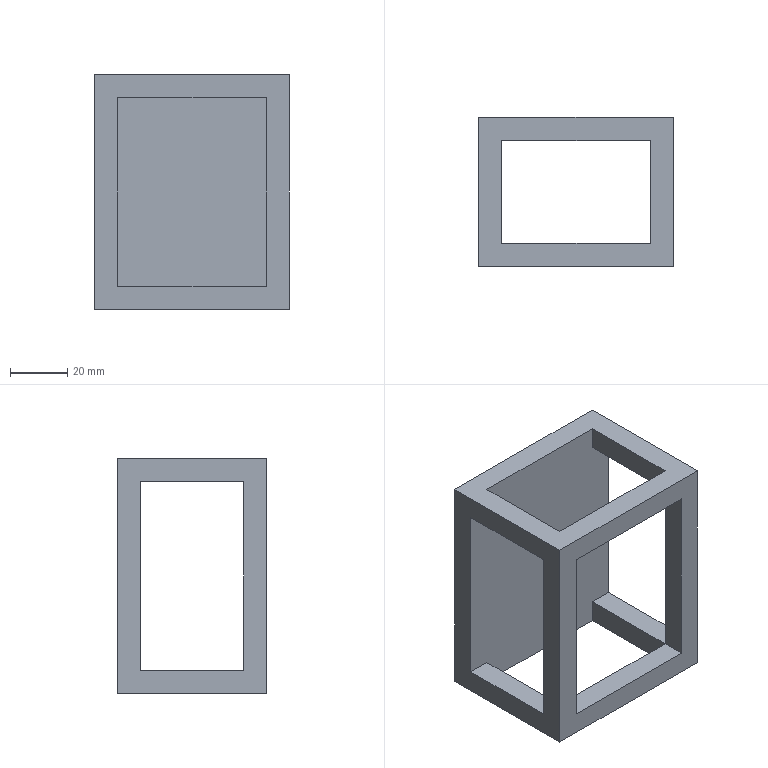Component | SolidWorks | MotorMount-1 | 1 solid | 23 faces | box 68 x 52 x 82 mm | volume 70976 mm3 | plane 23
build123d program:
from build123d import *

# Parameters (mm, degrees)
SKETCH1_W           = 82
SKETCH1_H           = 68
BOSS_EXTRUDE1_DEPTH = 52
SKETCH2_W           = 36
SKETCH2_H           = 52
CUT_EXTRUDE1_DEPTH  = 82
CUT_EXTRUDE2_REACH  = 96.916
SKETCH3_W           = 66
SKETCH3_H           = 36
SKETCH4_W           = 66
SKETCH4_H           = 52
CUT_EXTRUDE3_DEPTH  = 44


with BuildPart() as part:
    # Sketch1 → Boss-Extrude1 (new body)
    with BuildSketch(Plane.XY):
        Rectangle(SKETCH1_W, SKETCH1_H)
    extrude(amount=BOSS_EXTRUDE1_DEPTH)

    # Sketch2 → Cut-Extrude1 (cut)
    with BuildSketch(Plane(origin=(41, 0, 0), x_dir=(0, 0, -1), z_dir=(1, 0, 0))):
        with Locations((-26, 0)):
            Rectangle(SKETCH2_W, SKETCH2_H)
    extrude(amount=-CUT_EXTRUDE1_DEPTH, mode=Mode.SUBTRACT)

    # Cut-Extrude2: up to this face of the body (flat: up to its plane)
    cut_extrude2_end = Plane(part.part.faces().sort_by_distance((0, -34, 26))[0])
    # Sketch3 → Cut-Extrude2 (cut, up to the picked face)
    with BuildSketch(Plane(origin=(0, 34, 0), x_dir=(1, 0, 0), z_dir=(0, 1, 0)), mode=Mode.PRIVATE) as cut_extrude2_sk1:
        with Locations((0, -26)):
            Rectangle(SKETCH3_W, SKETCH3_H)
    cut_extrude2_tool1 = split(extrude(cut_extrude2_sk1.sketch, amount=-CUT_EXTRUDE2_REACH, mode=Mode.PRIVATE), bisect_by=cut_extrude2_end, keep=Keep.BOTH, mode=Mode.PRIVATE)
    add(cut_extrude2_tool1.solids().sort_by(Axis((0, 34, 26), (0, -1, 0)))[0], mode=Mode.SUBTRACT)

    # Sketch4 → Cut-Extrude3 (cut)
    with BuildSketch(Plane.XY.offset(52)):
        Rectangle(SKETCH4_W, SKETCH4_H)
    extrude(amount=-CUT_EXTRUDE3_DEPTH, mode=Mode.SUBTRACT)


solid = part.part

# Placed as in the assembly
solid = solid.moved(Location((-613.2, 52, 0), (90, 0, 90)))
STEP:
#1=CARTESIAN_POINT('',(-25.165,0.315,1.299));
#2=VERTEX_POINT('',#1);
#3=CARTESIAN_POINT('',(-25.48,0.315,1.299));
#4=VERTEX_POINT('',#3);
#5=CARTESIAN_POINT('',(-19.843,0.315,1.299));
#6=DIRECTION('',(-1.,0.,0.));
#7=VECTOR('',#6,39.37);
#8=LINE('',#5,#7);
#9=EDGE_CURVE('',#2,#4,#8,.T.);
#10=ORIENTED_EDGE('',*,*,#9,.F.);
#11=CARTESIAN_POINT('',(-25.165,0.315,-1.299));
#12=VERTEX_POINT('',#11);
#13=CARTESIAN_POINT('',(-25.165,0.315,-4.104));
#14=DIRECTION('',(-0.,0.,-1.));
#15=VECTOR('',#14,39.37);
#16=LINE('',#13,#15);
#17=EDGE_CURVE('',#2,#12,#16,.T.);
#18=ORIENTED_EDGE('',*,*,#17,.T.);
#19=CARTESIAN_POINT('',(-25.48,0.315,-1.299));
#20=VERTEX_POINT('',#19);
#21=CARTESIAN_POINT('',(-19.843,0.315,-1.299));
#22=DIRECTION('',(-1.,0.,0.));
#23=VECTOR('',#22,39.37);
#24=LINE('',#21,#23);
#25=EDGE_CURVE('',#12,#20,#24,.T.);
#26=ORIENTED_EDGE('',*,*,#25,.T.);
#27=CARTESIAN_POINT('',(-25.48,0.315,-1.299));
#28=DIRECTION('',(0.,-0.,1.));
#29=VECTOR('',#28,39.37);
#30=LINE('',#27,#29);
#31=EDGE_CURVE('',#20,#4,#30,.T.);
#32=ORIENTED_EDGE('',*,*,#31,.T.);
#33=EDGE_LOOP('',(#10,#18,#26,#32));
#34=FACE_OUTER_BOUND('',#33,.T.);
#35=CARTESIAN_POINT('',(-25.165,0.315,-4.104));
#36=DIRECTION('',(-0.,-1.,-0.));
#37=DIRECTION('',(0.,-0.,1.));
#38=AXIS2_PLACEMENT_3D('',#35,#36,#37);
#39=PLANE('',#38);
#40=ADVANCED_FACE('',(#34),#39,.F.);
#41=CARTESIAN_POINT('',(-25.165,0.315,-1.614));
#42=VERTEX_POINT('',#41);
#43=CARTESIAN_POINT('',(-25.165,0.315,-4.104));
#44=DIRECTION('',(0.,-0.,1.));
#45=VECTOR('',#44,39.37);
#46=LINE('',#43,#45);
#47=EDGE_CURVE('',#42,#12,#46,.T.);
#48=ORIENTED_EDGE('',*,*,#47,.T.);
#49=CARTESIAN_POINT('',(-23.118,0.315,-1.299));
#50=VERTEX_POINT('',#49);
#51=CARTESIAN_POINT('',(-25.165,0.315,-1.299));
#52=DIRECTION('',(1.,0.,-0.));
#53=VECTOR('',#52,39.37);
#54=LINE('',#51,#53);
#55=EDGE_CURVE('',#12,#50,#54,.T.);
#56=ORIENTED_EDGE('',*,*,#55,.T.);
#57=CARTESIAN_POINT('',(-23.118,0.315,-1.614));
#58=VERTEX_POINT('',#57);
#59=CARTESIAN_POINT('',(-23.118,0.315,-4.104));
#60=DIRECTION('',(0.,-0.,1.));
#61=VECTOR('',#60,39.37);
#62=LINE('',#59,#61);
#63=EDGE_CURVE('',#58,#50,#62,.T.);
#64=ORIENTED_EDGE('',*,*,#63,.F.);
#65=CARTESIAN_POINT('',(-25.165,0.315,-1.614));
#66=DIRECTION('',(-1.,0.,0.));
#67=VECTOR('',#66,39.37);
#68=LINE('',#65,#67);
#69=EDGE_CURVE('',#58,#42,#68,.T.);
#70=ORIENTED_EDGE('',*,*,#69,.T.);
#71=EDGE_LOOP('',(#48,#56,#64,#70));
#72=FACE_OUTER_BOUND('',#71,.T.);
#73=CARTESIAN_POINT('',(-25.165,0.315,-4.104));
#74=DIRECTION('',(-0.,-1.,-0.));
#75=DIRECTION('',(0.,-0.,1.));
#76=AXIS2_PLACEMENT_3D('',#73,#74,#75);
#77=PLANE('',#76);
#78=ADVANCED_FACE('',(#72),#77,.F.);
#79=CARTESIAN_POINT('',(-22.803,0.315,-1.299));
#80=VERTEX_POINT('',#79);
#81=CARTESIAN_POINT('',(-19.843,0.315,-1.299));
#82=DIRECTION('',(-1.,0.,0.));
#83=VECTOR('',#82,39.37);
#84=LINE('',#81,#83);
#85=EDGE_CURVE('',#80,#50,#84,.T.);
#86=ORIENTED_EDGE('',*,*,#85,.T.);
#87=CARTESIAN_POINT('',(-23.118,0.315,1.299));
#88=VERTEX_POINT('',#87);
#89=CARTESIAN_POINT('',(-23.118,0.315,-4.104));
#90=DIRECTION('',(0.,-0.,1.));
#91=VECTOR('',#90,39.37);
#92=LINE('',#89,#91);
#93=EDGE_CURVE('',#50,#88,#92,.T.);
#94=ORIENTED_EDGE('',*,*,#93,.T.);
#95=CARTESIAN_POINT('',(-22.803,0.315,1.299));
#96=VERTEX_POINT('',#95);
#97=CARTESIAN_POINT('',(-19.843,0.315,1.299));
#98=DIRECTION('',(-1.,0.,0.));
#99=VECTOR('',#98,39.37);
#100=LINE('',#97,#99);
#101=EDGE_CURVE('',#96,#88,#100,.T.);
#102=ORIENTED_EDGE('',*,*,#101,.F.);
#103=CARTESIAN_POINT('',(-22.803,0.315,-1.299));
#104=DIRECTION('',(-0.,0.,-1.));
#105=VECTOR('',#104,39.37);
#106=LINE('',#103,#105);
#107=EDGE_CURVE('',#96,#80,#106,.T.);
#108=ORIENTED_EDGE('',*,*,#107,.T.);
#109=EDGE_LOOP('',(#86,#94,#102,#108));
#110=FACE_OUTER_BOUND('',#109,.T.);
#111=CARTESIAN_POINT('',(-25.165,0.315,-4.104));
#112=DIRECTION('',(-0.,-1.,-0.));
#113=DIRECTION('',(0.,-0.,1.));
#114=AXIS2_PLACEMENT_3D('',#111,#112,#113);
#115=PLANE('',#114);
#116=ADVANCED_FACE('',(#110),#115,.F.);
#117=CARTESIAN_POINT('',(-23.118,1.732,1.299));
#118=VERTEX_POINT('',#117);
#119=CARTESIAN_POINT('',(-23.118,1.732,1.614));
#120=VERTEX_POINT('',#119);
#121=CARTESIAN_POINT('',(-23.118,1.732,-4.104));
#122=DIRECTION('',(0.,-0.,1.));
#123=VECTOR('',#122,39.37);
#124=LINE('',#121,#123);
#125=EDGE_CURVE('',#118,#120,#124,.T.);
#126=ORIENTED_EDGE('',*,*,#125,.F.);
#127=CARTESIAN_POINT('',(-23.118,0.315,1.299));
#128=DIRECTION('',(-0.,-1.,-0.));
#129=VECTOR('',#128,39.37);
#130=LINE('',#127,#129);
#131=EDGE_CURVE('',#118,#88,#130,.T.);
#132=ORIENTED_EDGE('',*,*,#131,.T.);
#133=CARTESIAN_POINT('',(-23.118,0.315,1.614));
#134=VERTEX_POINT('',#133);
#135=CARTESIAN_POINT('',(-23.118,0.315,-4.104));
#136=DIRECTION('',(0.,-0.,1.));
#137=VECTOR('',#136,39.37);
#138=LINE('',#135,#137);
#139=EDGE_CURVE('',#88,#134,#138,.T.);
#140=ORIENTED_EDGE('',*,*,#139,.T.);
#141=CARTESIAN_POINT('',(-23.118,0.315,1.614));
#142=DIRECTION('',(0.,1.,0.));
#143=VECTOR('',#142,39.37);
#144=LINE('',#141,#143);
#145=EDGE_CURVE('',#134,#120,#144,.T.);
#146=ORIENTED_EDGE('',*,*,#145,.T.);
#147=EDGE_LOOP('',(#126,#132,#140,#146));
#148=FACE_OUTER_BOUND('',#147,.T.);
#149=CARTESIAN_POINT('',(-23.118,0.315,-4.104));
#150=DIRECTION('',(1.,-0.,-0.));
#151=DIRECTION('',(0.,1.,0.));
#152=AXIS2_PLACEMENT_3D('',#149,#150,#151);
#153=PLANE('',#152);
#154=ADVANCED_FACE('',(#148),#153,.F.);
#155=CARTESIAN_POINT('',(-25.165,0.315,1.614));
#156=VERTEX_POINT('',#155);
#157=CARTESIAN_POINT('',(-25.165,0.315,-4.104));
#158=DIRECTION('',(0.,-0.,1.));
#159=VECTOR('',#158,39.37);
#160=LINE('',#157,#159);
#161=EDGE_CURVE('',#2,#156,#160,.T.);
#162=ORIENTED_EDGE('',*,*,#161,.F.);
#163=CARTESIAN_POINT('',(-25.165,1.732,1.299));
#164=VERTEX_POINT('',#163);
#165=CARTESIAN_POINT('',(-25.165,1.732,1.299));
#166=DIRECTION('',(0.,1.,0.));
#167=VECTOR('',#166,39.37);
#168=LINE('',#165,#167);
#169=EDGE_CURVE('',#2,#164,#168,.T.);
#170=ORIENTED_EDGE('',*,*,#169,.T.);
#171=CARTESIAN_POINT('',(-25.165,1.732,1.614));
#172=VERTEX_POINT('',#171);
#173=CARTESIAN_POINT('',(-25.165,1.732,-4.104));
#174=DIRECTION('',(0.,-0.,1.));
#175=VECTOR('',#174,39.37);
#176=LINE('',#173,#175);
#177=EDGE_CURVE('',#164,#172,#176,.T.);
#178=ORIENTED_EDGE('',*,*,#177,.T.);
#179=CARTESIAN_POINT('',(-25.165,1.732,1.614));
#180=DIRECTION('',(-0.,-1.,-0.));
#181=VECTOR('',#180,39.37);
#182=LINE('',#179,#181);
#183=EDGE_CURVE('',#172,#156,#182,.T.);
#184=ORIENTED_EDGE('',*,*,#183,.T.);
#185=EDGE_LOOP('',(#162,#170,#178,#184));
#186=FACE_OUTER_BOUND('',#185,.T.);
#187=CARTESIAN_POINT('',(-25.165,1.732,-4.104));
#188=DIRECTION('',(-1.,0.,0.));
#189=DIRECTION('',(-0.,-1.,-0.));
#190=AXIS2_PLACEMENT_3D('',#187,#188,#189);
#191=PLANE('',#190);
#192=ADVANCED_FACE('',(#186),#191,.F.);
#193=CARTESIAN_POINT('',(-22.803,2.047,1.614));
#194=VERTEX_POINT('',#193);
#195=CARTESIAN_POINT('',(-25.48,2.047,1.614));
#196=VERTEX_POINT('',#195);
#197=CARTESIAN_POINT('',(-22.803,2.047,1.614));
#198=DIRECTION('',(-1.,0.,0.));
#199=VECTOR('',#198,39.37);
#200=LINE('',#197,#199);
#201=EDGE_CURVE('',#194,#196,#200,.T.);
#202=ORIENTED_EDGE('',*,*,#201,.F.);
#203=CARTESIAN_POINT('',(-22.803,2.047,-1.614));
#204=VERTEX_POINT('',#203);
#205=CARTESIAN_POINT('',(-22.803,2.047,1.614));
#206=DIRECTION('',(0.,-0.,1.));
#207=VECTOR('',#206,39.37);
#208=LINE('',#205,#207);
#209=EDGE_CURVE('',#204,#194,#208,.T.);
#210=ORIENTED_EDGE('',*,*,#209,.F.);
#211=CARTESIAN_POINT('',(-25.48,2.047,-1.614));
#212=VERTEX_POINT('',#211);
#213=CARTESIAN_POINT('',(-22.803,2.047,-1.614));
#214=DIRECTION('',(1.,0.,-0.));
#215=VECTOR('',#214,39.37);
#216=LINE('',#213,#215);
#217=EDGE_CURVE('',#212,#204,#216,.T.);
#218=ORIENTED_EDGE('',*,*,#217,.F.);
#219=CARTESIAN_POINT('',(-25.48,2.047,1.614));
#220=DIRECTION('',(-0.,0.,-1.));
#221=VECTOR('',#220,39.37);
#222=LINE('',#219,#221);
#223=EDGE_CURVE('',#196,#212,#222,.T.);
#224=ORIENTED_EDGE('',*,*,#223,.F.);
#225=EDGE_LOOP('',(#202,#210,#218,#224));
#226=FACE_OUTER_BOUND('',#225,.T.);
#227=CARTESIAN_POINT('',(-24.142,2.047,0.));
#228=DIRECTION('',(-0.,-1.,-0.));
#229=DIRECTION('',(0.,-0.,1.));
#230=AXIS2_PLACEMENT_3D('',#227,#228,#229);
#231=PLANE('',#230);
#232=ADVANCED_FACE('',(#226),#231,.F.);
#233=CARTESIAN_POINT('',(-22.803,1.732,1.299));
#234=VERTEX_POINT('',#233);
#235=CARTESIAN_POINT('',(-22.803,0.315,1.299));
#236=DIRECTION('',(-0.,-1.,-0.));
#237=VECTOR('',#236,39.37);
#238=LINE('',#235,#237);
#239=EDGE_CURVE('',#234,#96,#238,.T.);
#240=ORIENTED_EDGE('',*,*,#239,.F.);
#241=CARTESIAN_POINT('',(-22.803,1.732,-1.299));
#242=VERTEX_POINT('',#241);
#243=CARTESIAN_POINT('',(-22.803,1.732,1.299));
#244=DIRECTION('',(0.,-0.,1.));
#245=VECTOR('',#244,39.37);
#246=LINE('',#243,#245);
#247=EDGE_CURVE('',#242,#234,#246,.T.);
#248=ORIENTED_EDGE('',*,*,#247,.F.);
#249=CARTESIAN_POINT('',(-22.803,1.732,-1.299));
#250=DIRECTION('',(0.,1.,0.));
#251=VECTOR('',#250,39.37);
#252=LINE('',#249,#251);
#253=EDGE_CURVE('',#80,#242,#252,.T.);
#254=ORIENTED_EDGE('',*,*,#253,.F.);
#255=ORIENTED_EDGE('',*,*,#107,.F.);
#256=EDGE_LOOP('',(#240,#248,#254,#255));
#257=FACE_BOUND('',#256,.T.);
#258=CARTESIAN_POINT('',(-22.803,-0.,1.614));
#259=VERTEX_POINT('',#258);
#260=CARTESIAN_POINT('',(-22.803,-4.194,1.614));
#261=DIRECTION('',(0.,1.,0.));
#262=VECTOR('',#261,39.37);
#263=LINE('',#260,#262);
#264=EDGE_CURVE('',#259,#194,#263,.T.);
#265=ORIENTED_EDGE('',*,*,#264,.F.);
#266=CARTESIAN_POINT('',(-22.803,0.,-1.614));
#267=VERTEX_POINT('',#266);
#268=CARTESIAN_POINT('',(-22.803,-0.,1.614));
#269=DIRECTION('',(-0.,0.,-1.));
#270=VECTOR('',#269,39.37);
#271=LINE('',#268,#270);
#272=EDGE_CURVE('',#259,#267,#271,.T.);
#273=ORIENTED_EDGE('',*,*,#272,.T.);
#274=CARTESIAN_POINT('',(-22.803,-4.194,-1.614));
#275=DIRECTION('',(0.,1.,0.));
#276=VECTOR('',#275,39.37);
#277=LINE('',#274,#276);
#278=EDGE_CURVE('',#267,#204,#277,.T.);
#279=ORIENTED_EDGE('',*,*,#278,.T.);
#280=ORIENTED_EDGE('',*,*,#209,.T.);
#281=EDGE_LOOP('',(#265,#273,#279,#280));
#282=FACE_OUTER_BOUND('',#281,.T.);
#283=CARTESIAN_POINT('',(-22.803,-4.194,1.614));
#284=DIRECTION('',(-1.,0.,0.));
#285=DIRECTION('',(-0.,-1.,-0.));
#286=AXIS2_PLACEMENT_3D('',#283,#284,#285);
#287=PLANE('',#286);
#288=ADVANCED_FACE('',(#257,#282),#287,.F.);
#289=CARTESIAN_POINT('',(-23.118,1.732,-1.614));
#290=VERTEX_POINT('',#289);
#291=CARTESIAN_POINT('',(-23.118,0.315,-1.614));
#292=DIRECTION('',(-0.,-1.,-0.));
#293=VECTOR('',#292,39.37);
#294=LINE('',#291,#293);
#295=EDGE_CURVE('',#290,#58,#294,.T.);
#296=ORIENTED_EDGE('',*,*,#295,.F.);
#297=CARTESIAN_POINT('',(-25.165,1.732,-1.614));
#298=VERTEX_POINT('',#297);
#299=CARTESIAN_POINT('',(-23.118,1.732,-1.614));
#300=DIRECTION('',(1.,0.,-0.));
#301=VECTOR('',#300,39.37);
#302=LINE('',#299,#301);
#303=EDGE_CURVE('',#298,#290,#302,.T.);
#304=ORIENTED_EDGE('',*,*,#303,.F.);
#305=CARTESIAN_POINT('',(-25.165,1.732,-1.614));
#306=DIRECTION('',(0.,1.,0.));
#307=VECTOR('',#306,39.37);
#308=LINE('',#305,#307);
#309=EDGE_CURVE('',#42,#298,#308,.T.);
#310=ORIENTED_EDGE('',*,*,#309,.F.);
#311=ORIENTED_EDGE('',*,*,#69,.F.);
#312=EDGE_LOOP('',(#296,#304,#310,#311));
#313=FACE_BOUND('',#312,.T.);
#314=ORIENTED_EDGE('',*,*,#278,.F.);
#315=CARTESIAN_POINT('',(-25.48,0.,-1.614));
#316=VERTEX_POINT('',#315);
#317=CARTESIAN_POINT('',(-22.803,0.,-1.614));
#318=DIRECTION('',(-1.,0.,0.));
#319=VECTOR('',#318,39.37);
#320=LINE('',#317,#319);
#321=EDGE_CURVE('',#267,#316,#320,.T.);
#322=ORIENTED_EDGE('',*,*,#321,.T.);
#323=CARTESIAN_POINT('',(-25.48,-4.194,-1.614));
#324=DIRECTION('',(0.,1.,0.));
#325=VECTOR('',#324,39.37);
#326=LINE('',#323,#325);
#327=EDGE_CURVE('',#316,#212,#326,.T.);
#328=ORIENTED_EDGE('',*,*,#327,.T.);
#329=ORIENTED_EDGE('',*,*,#217,.T.);
#330=EDGE_LOOP('',(#314,#322,#328,#329));
#331=FACE_OUTER_BOUND('',#330,.T.);
#332=CARTESIAN_POINT('',(-22.803,-4.194,-1.614));
#333=DIRECTION('',(0.,-0.,1.));
#334=DIRECTION('',(0.,1.,0.));
#335=AXIS2_PLACEMENT_3D('',#332,#333,#334);
#336=PLANE('',#335);
#337=ADVANCED_FACE('',(#313,#331),#336,.F.);
#338=CARTESIAN_POINT('',(-25.48,1.732,-1.299));
#339=VERTEX_POINT('',#338);
#340=CARTESIAN_POINT('',(-25.48,1.732,-1.299));
#341=DIRECTION('',(-0.,-1.,-0.));
#342=VECTOR('',#341,39.37);
#343=LINE('',#340,#342);
#344=EDGE_CURVE('',#339,#20,#343,.T.);
#345=ORIENTED_EDGE('',*,*,#344,.F.);
#346=CARTESIAN_POINT('',(-25.48,1.732,1.299));
#347=VERTEX_POINT('',#346);
#348=CARTESIAN_POINT('',(-25.48,1.732,1.299));
#349=DIRECTION('',(-0.,0.,-1.));
#350=VECTOR('',#349,39.37);
#351=LINE('',#348,#350);
#352=EDGE_CURVE('',#347,#339,#351,.T.);
#353=ORIENTED_EDGE('',*,*,#352,.F.);
#354=CARTESIAN_POINT('',(-25.48,0.315,1.299));
#355=DIRECTION('',(0.,1.,0.));
#356=VECTOR('',#355,39.37);
#357=LINE('',#354,#356);
#358=EDGE_CURVE('',#4,#347,#357,.T.);
#359=ORIENTED_EDGE('',*,*,#358,.F.);
#360=ORIENTED_EDGE('',*,*,#31,.F.);
#361=EDGE_LOOP('',(#345,#353,#359,#360));
#362=FACE_BOUND('',#361,.T.);
#363=ORIENTED_EDGE('',*,*,#327,.F.);
#364=CARTESIAN_POINT('',(-25.48,-0.,1.614));
#365=VERTEX_POINT('',#364);
#366=CARTESIAN_POINT('',(-25.48,-0.,1.614));
#367=DIRECTION('',(0.,0.,1.));
#368=VECTOR('',#367,39.37);
#369=LINE('',#366,#368);
#370=EDGE_CURVE('',#316,#365,#369,.T.);
#371=ORIENTED_EDGE('',*,*,#370,.T.);
#372=CARTESIAN_POINT('',(-25.48,-4.194,1.614));
#373=DIRECTION('',(0.,1.,0.));
#374=VECTOR('',#373,39.37);
#375=LINE('',#372,#374);
#376=EDGE_CURVE('',#365,#196,#375,.T.);
#377=ORIENTED_EDGE('',*,*,#376,.T.);
#378=ORIENTED_EDGE('',*,*,#223,.T.);
#379=EDGE_LOOP('',(#363,#371,#377,#378));
#380=FACE_OUTER_BOUND('',#379,.T.);
#381=CARTESIAN_POINT('',(-25.48,-4.194,1.614));
#382=DIRECTION('',(1.,-0.,-0.));
#383=DIRECTION('',(0.,1.,0.));
#384=AXIS2_PLACEMENT_3D('',#381,#382,#383);
#385=PLANE('',#384);
#386=ADVANCED_FACE('',(#362,#380),#385,.F.);
#387=ORIENTED_EDGE('',*,*,#183,.F.);
#388=CARTESIAN_POINT('',(-23.118,1.732,1.614));
#389=DIRECTION('',(-1.,0.,0.));
#390=VECTOR('',#389,39.37);
#391=LINE('',#388,#390);
#392=EDGE_CURVE('',#120,#172,#391,.T.);
#393=ORIENTED_EDGE('',*,*,#392,.F.);
#394=ORIENTED_EDGE('',*,*,#145,.F.);
#395=CARTESIAN_POINT('',(-25.165,0.315,1.614));
#396=DIRECTION('',(1.,0.,-0.));
#397=VECTOR('',#396,39.37);
#398=LINE('',#395,#397);
#399=EDGE_CURVE('',#156,#134,#398,.T.);
#400=ORIENTED_EDGE('',*,*,#399,.F.);
#401=EDGE_LOOP('',(#387,#393,#394,#400));
#402=FACE_BOUND('',#401,.T.);
#403=ORIENTED_EDGE('',*,*,#376,.F.);
#404=CARTESIAN_POINT('',(-22.803,-0.,1.614));
#405=DIRECTION('',(1.,0.,-0.));
#406=VECTOR('',#405,39.37);
#407=LINE('',#404,#406);
#408=EDGE_CURVE('',#365,#259,#407,.T.);
#409=ORIENTED_EDGE('',*,*,#408,.T.);
#410=ORIENTED_EDGE('',*,*,#264,.T.);
#411=ORIENTED_EDGE('',*,*,#201,.T.);
#412=EDGE_LOOP('',(#403,#409,#410,#411));
#413=FACE_OUTER_BOUND('',#412,.T.);
#414=CARTESIAN_POINT('',(-22.803,-4.194,1.614));
#415=DIRECTION('',(-0.,0.,-1.));
#416=DIRECTION('',(-0.,-1.,-0.));
#417=AXIS2_PLACEMENT_3D('',#414,#415,#416);
#418=PLANE('',#417);
#419=ADVANCED_FACE('',(#402,#413),#418,.F.);
#420=CARTESIAN_POINT('',(-25.165,0.,-1.299));
#421=VERTEX_POINT('',#420);
#422=CARTESIAN_POINT('',(-23.118,0.,-1.299));
#423=VERTEX_POINT('',#422);
#424=CARTESIAN_POINT('',(-25.165,0.,-1.299));
#425=DIRECTION('',(1.,0.,-0.));
#426=VECTOR('',#425,39.37);
#427=LINE('',#424,#426);
#428=EDGE_CURVE('',#421,#423,#427,.T.);
#429=ORIENTED_EDGE('',*,*,#428,.F.);
#430=CARTESIAN_POINT('',(-25.165,-0.,1.299));
#431=VERTEX_POINT('',#430);
#432=CARTESIAN_POINT('',(-25.165,-0.,1.299));
#433=DIRECTION('',(-0.,0.,-1.));
#434=VECTOR('',#433,39.37);
#435=LINE('',#432,#434);
#436=EDGE_CURVE('',#431,#421,#435,.T.);
#437=ORIENTED_EDGE('',*,*,#436,.F.);
#438=CARTESIAN_POINT('',(-23.118,0.,1.299));
#439=VERTEX_POINT('',#438);
#440=CARTESIAN_POINT('',(-23.118,-0.,1.299));
#441=DIRECTION('',(-1.,0.,0.));
#442=VECTOR('',#441,39.37);
#443=LINE('',#440,#442);
#444=EDGE_CURVE('',#439,#431,#443,.T.);
#445=ORIENTED_EDGE('',*,*,#444,.F.);
#446=CARTESIAN_POINT('',(-23.118,0.,-1.299));
#447=DIRECTION('',(0.,-0.,1.));
#448=VECTOR('',#447,39.37);
#449=LINE('',#446,#448);
#450=EDGE_CURVE('',#423,#439,#449,.T.);
#451=ORIENTED_EDGE('',*,*,#450,.F.);
#452=EDGE_LOOP('',(#429,#437,#445,#451));
#453=FACE_BOUND('',#452,.T.);
#454=ORIENTED_EDGE('',*,*,#370,.F.);
#455=ORIENTED_EDGE('',*,*,#321,.F.);
#456=ORIENTED_EDGE('',*,*,#272,.F.);
#457=ORIENTED_EDGE('',*,*,#408,.F.);
#458=EDGE_LOOP('',(#454,#455,#456,#457));
#459=FACE_OUTER_BOUND('',#458,.T.);
#460=CARTESIAN_POINT('',(0.,0.,-0.));
#461=DIRECTION('',(-0.,1.,-0.));
#462=DIRECTION('',(1.,0.,0.));
#463=AXIS2_PLACEMENT_3D('',#460,#461,#462);
#464=PLANE('',#463);
#465=ADVANCED_FACE('',(#453,#459),#464,.F.);
#466=ORIENTED_EDGE('',*,*,#177,.F.);
#467=CARTESIAN_POINT('',(-19.843,1.732,1.299));
#468=DIRECTION('',(-1.,0.,0.));
#469=VECTOR('',#468,39.37);
#470=LINE('',#467,#469);
#471=EDGE_CURVE('',#164,#347,#470,.T.);
#472=ORIENTED_EDGE('',*,*,#471,.T.);
#473=ORIENTED_EDGE('',*,*,#352,.T.);
#474=CARTESIAN_POINT('',(-25.165,1.732,-1.299));
#475=VERTEX_POINT('',#474);
#476=CARTESIAN_POINT('',(-19.843,1.732,-1.299));
#477=DIRECTION('',(-1.,0.,0.));
#478=VECTOR('',#477,39.37);
#479=LINE('',#476,#478);
#480=EDGE_CURVE('',#475,#339,#479,.T.);
#481=ORIENTED_EDGE('',*,*,#480,.F.);
#482=CARTESIAN_POINT('',(-25.165,1.732,-4.104));
#483=DIRECTION('',(0.,-0.,1.));
#484=VECTOR('',#483,39.37);
#485=LINE('',#482,#484);
#486=EDGE_CURVE('',#298,#475,#485,.T.);
#487=ORIENTED_EDGE('',*,*,#486,.F.);
#488=ORIENTED_EDGE('',*,*,#303,.T.);
#489=CARTESIAN_POINT('',(-23.118,1.732,-1.299));
#490=VERTEX_POINT('',#489);
#491=CARTESIAN_POINT('',(-23.118,1.732,-4.104));
#492=DIRECTION('',(0.,-0.,1.));
#493=VECTOR('',#492,39.37);
#494=LINE('',#491,#493);
#495=EDGE_CURVE('',#290,#490,#494,.T.);
#496=ORIENTED_EDGE('',*,*,#495,.T.);
#497=CARTESIAN_POINT('',(-19.843,1.732,-1.299));
#498=DIRECTION('',(-1.,0.,0.));
#499=VECTOR('',#498,39.37);
#500=LINE('',#497,#499);
#501=EDGE_CURVE('',#242,#490,#500,.T.);
#502=ORIENTED_EDGE('',*,*,#501,.F.);
#503=ORIENTED_EDGE('',*,*,#247,.T.);
#504=CARTESIAN_POINT('',(-19.843,1.732,1.299));
#505=DIRECTION('',(-1.,0.,0.));
#506=VECTOR('',#505,39.37);
#507=LINE('',#504,#506);
#508=EDGE_CURVE('',#234,#118,#507,.T.);
#509=ORIENTED_EDGE('',*,*,#508,.T.);
#510=ORIENTED_EDGE('',*,*,#125,.T.);
#511=ORIENTED_EDGE('',*,*,#392,.T.);
#512=EDGE_LOOP('',(#466,#472,#473,#481,#487,#488,#496,#502,#503,#509,#510,#511));
#513=FACE_OUTER_BOUND('',#512,.T.);
#514=CARTESIAN_POINT('',(-23.118,1.732,-4.104));
#515=DIRECTION('',(0.,1.,0.));
#516=DIRECTION('',(-0.,0.,-1.));
#517=AXIS2_PLACEMENT_3D('',#514,#515,#516);
#518=PLANE('',#517);
#519=ADVANCED_FACE('',(#513),#518,.F.);
#520=ORIENTED_EDGE('',*,*,#63,.T.);
#521=CARTESIAN_POINT('',(-23.118,0.315,-1.299));
#522=DIRECTION('',(0.,1.,0.));
#523=VECTOR('',#522,39.37);
#524=LINE('',#521,#523);
#525=EDGE_CURVE('',#50,#490,#524,.T.);
#526=ORIENTED_EDGE('',*,*,#525,.T.);
#527=ORIENTED_EDGE('',*,*,#495,.F.);
#528=ORIENTED_EDGE('',*,*,#295,.T.);
#529=EDGE_LOOP('',(#520,#526,#527,#528));
#530=FACE_OUTER_BOUND('',#529,.T.);
#531=CARTESIAN_POINT('',(-23.118,0.315,-4.104));
#532=DIRECTION('',(1.,-0.,-0.));
#533=DIRECTION('',(0.,1.,0.));
#534=AXIS2_PLACEMENT_3D('',#531,#532,#533);
#535=PLANE('',#534);
#536=ADVANCED_FACE('',(#530),#535,.F.);
#537=ORIENTED_EDGE('',*,*,#139,.F.);
#538=CARTESIAN_POINT('',(-25.165,0.315,1.299));
#539=DIRECTION('',(-1.,0.,0.));
#540=VECTOR('',#539,39.37);
#541=LINE('',#538,#540);
#542=EDGE_CURVE('',#88,#2,#541,.T.);
#543=ORIENTED_EDGE('',*,*,#542,.T.);
#544=ORIENTED_EDGE('',*,*,#161,.T.);
#545=ORIENTED_EDGE('',*,*,#399,.T.);
#546=EDGE_LOOP('',(#537,#543,#544,#545));
#547=FACE_OUTER_BOUND('',#546,.T.);
#548=CARTESIAN_POINT('',(-25.165,0.315,-4.104));
#549=DIRECTION('',(-0.,-1.,-0.));
#550=DIRECTION('',(0.,-0.,1.));
#551=AXIS2_PLACEMENT_3D('',#548,#549,#550);
#552=PLANE('',#551);
#553=ADVANCED_FACE('',(#547),#552,.F.);
#554=ORIENTED_EDGE('',*,*,#486,.T.);
#555=CARTESIAN_POINT('',(-25.165,1.732,-1.299));
#556=DIRECTION('',(-0.,-1.,-0.));
#557=VECTOR('',#556,39.37);
#558=LINE('',#555,#557);
#559=EDGE_CURVE('',#475,#12,#558,.T.);
#560=ORIENTED_EDGE('',*,*,#559,.T.);
#561=ORIENTED_EDGE('',*,*,#47,.F.);
#562=ORIENTED_EDGE('',*,*,#309,.T.);
#563=EDGE_LOOP('',(#554,#560,#561,#562));
#564=FACE_OUTER_BOUND('',#563,.T.);
#565=CARTESIAN_POINT('',(-25.165,1.732,-4.104));
#566=DIRECTION('',(-1.,0.,0.));
#567=DIRECTION('',(-0.,-1.,-0.));
#568=AXIS2_PLACEMENT_3D('',#565,#566,#567);
#569=PLANE('',#568);
#570=ADVANCED_FACE('',(#564),#569,.F.);
#571=ORIENTED_EDGE('',*,*,#480,.T.);
#572=ORIENTED_EDGE('',*,*,#344,.T.);
#573=ORIENTED_EDGE('',*,*,#25,.F.);
#574=ORIENTED_EDGE('',*,*,#559,.F.);
#575=EDGE_LOOP('',(#571,#572,#573,#574));
#576=FACE_OUTER_BOUND('',#575,.T.);
#577=CARTESIAN_POINT('',(-19.843,1.732,-1.299));
#578=DIRECTION('',(-0.,0.,-1.));
#579=DIRECTION('',(-0.,-1.,-0.));
#580=AXIS2_PLACEMENT_3D('',#577,#578,#579);
#581=PLANE('',#580);
#582=ADVANCED_FACE('',(#576),#581,.F.);
#583=ORIENTED_EDGE('',*,*,#9,.T.);
#584=ORIENTED_EDGE('',*,*,#358,.T.);
#585=ORIENTED_EDGE('',*,*,#471,.F.);
#586=ORIENTED_EDGE('',*,*,#169,.F.);
#587=EDGE_LOOP('',(#583,#584,#585,#586));
#588=FACE_OUTER_BOUND('',#587,.T.);
#589=CARTESIAN_POINT('',(-19.843,0.315,1.299));
#590=DIRECTION('',(0.,-0.,1.));
#591=DIRECTION('',(0.,1.,0.));
#592=AXIS2_PLACEMENT_3D('',#589,#590,#591);
#593=PLANE('',#592);
#594=ADVANCED_FACE('',(#588),#593,.F.);
#595=ORIENTED_EDGE('',*,*,#508,.F.);
#596=ORIENTED_EDGE('',*,*,#239,.T.);
#597=ORIENTED_EDGE('',*,*,#101,.T.);
#598=ORIENTED_EDGE('',*,*,#131,.F.);
#599=EDGE_LOOP('',(#595,#596,#597,#598));
#600=FACE_OUTER_BOUND('',#599,.T.);
#601=CARTESIAN_POINT('',(-19.843,0.315,1.299));
#602=DIRECTION('',(0.,-0.,1.));
#603=DIRECTION('',(0.,1.,0.));
#604=AXIS2_PLACEMENT_3D('',#601,#602,#603);
#605=PLANE('',#604);
#606=ADVANCED_FACE('',(#600),#605,.F.);
#607=ORIENTED_EDGE('',*,*,#85,.F.);
#608=ORIENTED_EDGE('',*,*,#253,.T.);
#609=ORIENTED_EDGE('',*,*,#501,.T.);
#610=ORIENTED_EDGE('',*,*,#525,.F.);
#611=EDGE_LOOP('',(#607,#608,#609,#610));
#612=FACE_OUTER_BOUND('',#611,.T.);
#613=CARTESIAN_POINT('',(-19.843,1.732,-1.299));
#614=DIRECTION('',(-0.,0.,-1.));
#615=DIRECTION('',(-0.,-1.,-0.));
#616=AXIS2_PLACEMENT_3D('',#613,#614,#615);
#617=PLANE('',#616);
#618=ADVANCED_FACE('',(#612),#617,.F.);
#619=CARTESIAN_POINT('',(-23.118,5.04,1.299));
#620=DIRECTION('',(-0.,-1.,-0.));
#621=VECTOR('',#620,39.37);
#622=LINE('',#619,#621);
#623=EDGE_CURVE('',#88,#439,#622,.T.);
#624=ORIENTED_EDGE('',*,*,#623,.T.);
#625=ORIENTED_EDGE('',*,*,#444,.T.);
#626=CARTESIAN_POINT('',(-25.165,5.04,1.299));
#627=DIRECTION('',(-0.,-1.,-0.));
#628=VECTOR('',#627,39.37);
#629=LINE('',#626,#628);
#630=EDGE_CURVE('',#2,#431,#629,.T.);
#631=ORIENTED_EDGE('',*,*,#630,.F.);
#632=ORIENTED_EDGE('',*,*,#542,.F.);
#633=EDGE_LOOP('',(#624,#625,#631,#632));
#634=FACE_OUTER_BOUND('',#633,.T.);
#635=CARTESIAN_POINT('',(-23.118,5.04,1.299));
#636=DIRECTION('',(0.,-0.,1.));
#637=DIRECTION('',(0.,1.,0.));
#638=AXIS2_PLACEMENT_3D('',#635,#636,#637);
#639=PLANE('',#638);
#640=ADVANCED_FACE('',(#634),#639,.F.);
#641=CARTESIAN_POINT('',(-25.165,5.04,-1.299));
#642=DIRECTION('',(-0.,-1.,-0.));
#643=VECTOR('',#642,39.37);
#644=LINE('',#641,#643);
#645=EDGE_CURVE('',#12,#421,#644,.T.);
#646=ORIENTED_EDGE('',*,*,#645,.T.);
#647=ORIENTED_EDGE('',*,*,#428,.T.);
#648=CARTESIAN_POINT('',(-23.118,5.04,-1.299));
#649=DIRECTION('',(-0.,-1.,-0.));
#650=VECTOR('',#649,39.37);
#651=LINE('',#648,#650);
#652=EDGE_CURVE('',#50,#423,#651,.T.);
#653=ORIENTED_EDGE('',*,*,#652,.F.);
#654=ORIENTED_EDGE('',*,*,#55,.F.);
#655=EDGE_LOOP('',(#646,#647,#653,#654));
#656=FACE_OUTER_BOUND('',#655,.T.);
#657=CARTESIAN_POINT('',(-25.165,5.04,-1.299));
#658=DIRECTION('',(-0.,0.,-1.));
#659=DIRECTION('',(-0.,-1.,-0.));
#660=AXIS2_PLACEMENT_3D('',#657,#658,#659);
#661=PLANE('',#660);
#662=ADVANCED_FACE('',(#656),#661,.F.);
#663=ORIENTED_EDGE('',*,*,#630,.T.);
#664=ORIENTED_EDGE('',*,*,#436,.T.);
#665=ORIENTED_EDGE('',*,*,#645,.F.);
#666=ORIENTED_EDGE('',*,*,#17,.F.);
#667=EDGE_LOOP('',(#663,#664,#665,#666));
#668=FACE_OUTER_BOUND('',#667,.T.);
#669=CARTESIAN_POINT('',(-25.165,5.04,1.299));
#670=DIRECTION('',(-1.,0.,0.));
#671=DIRECTION('',(-0.,0.,-1.));
#672=AXIS2_PLACEMENT_3D('',#669,#670,#671);
#673=PLANE('',#672);
#674=ADVANCED_FACE('',(#668),#673,.F.);
#675=ORIENTED_EDGE('',*,*,#652,.T.);
#676=ORIENTED_EDGE('',*,*,#450,.T.);
#677=ORIENTED_EDGE('',*,*,#623,.F.);
#678=ORIENTED_EDGE('',*,*,#93,.F.);
#679=EDGE_LOOP('',(#675,#676,#677,#678));
#680=FACE_OUTER_BOUND('',#679,.T.);
#681=CARTESIAN_POINT('',(-23.118,5.04,-1.299));
#682=DIRECTION('',(1.,-0.,-0.));
#683=DIRECTION('',(0.,1.,0.));
#684=AXIS2_PLACEMENT_3D('',#681,#682,#683);
#685=PLANE('',#684);
#686=ADVANCED_FACE('',(#680),#685,.F.);
#687=CLOSED_SHELL('',(#40,#78,#116,#154,#192,#232,#288,#337,#386,#419,#465,#519,#536,#553,#570,#582,#594,#606,#618,#640,#662,#674,#686));
#688=MANIFOLD_SOLID_BREP('',#687);
#689=CARTESIAN_POINT('',(0.,0.,0.));
#690=DIRECTION('',(0.,0.,1.));
#691=DIRECTION('',(1.,0.,0.));
#692=AXIS2_PLACEMENT_3D('',#689,#690,#691);
#693=(LENGTH_UNIT()NAMED_UNIT(*)SI_UNIT($,.METRE.));
#694=LENGTH_MEASURE_WITH_UNIT(LENGTH_MEASURE(0.0254),#693);
#695=DIMENSIONAL_EXPONENTS(1.,0.,0.,0.,0.,0.,0.);
#696=(CONVERSION_BASED_UNIT('',#694)LENGTH_UNIT()NAMED_UNIT(#695));
#697=UNCERTAINTY_MEASURE_WITH_UNIT(LENGTH_MEASURE(0.00001),#696,'','');
#698=(NAMED_UNIT(*)PLANE_ANGLE_UNIT()SI_UNIT($,.RADIAN.));
#699=(NAMED_UNIT(*)SI_UNIT($,.STERADIAN.)SOLID_ANGLE_UNIT());
#700=(GEOMETRIC_REPRESENTATION_CONTEXT(3)GLOBAL_UNCERTAINTY_ASSIGNED_CONTEXT((#697))GLOBAL_UNIT_ASSIGNED_CONTEXT((#696,#698,#699))REPRESENTATION_CONTEXT('',''));
#701=ADVANCED_BREP_SHAPE_REPRESENTATION('',(#688,#692),#700);
#702=COLOUR_RGB('',0.7922,0.8196,0.9333);
#703=FILL_AREA_STYLE_COLOUR('',#702);
#704=FILL_AREA_STYLE('',(#703));
#705=SURFACE_STYLE_FILL_AREA(#704);
#706=SURFACE_SIDE_STYLE('',(#705));
#707=SURFACE_STYLE_USAGE(.BOTH.,#706);
#708=PRESENTATION_STYLE_ASSIGNMENT((#707));
#709=STYLED_ITEM('',(#708),#688);
#710=PRESENTATION_LAYER_ASSIGNMENT('','',(#709));
#711=(LENGTH_UNIT()NAMED_UNIT(*)SI_UNIT($,.METRE.));
#712=LENGTH_MEASURE_WITH_UNIT(LENGTH_MEASURE(0.0254),#711);
#713=DIMENSIONAL_EXPONENTS(1.,0.,0.,0.,0.,0.,0.);
#714=(CONVERSION_BASED_UNIT('',#712)LENGTH_UNIT()NAMED_UNIT(#713));
#715=UNCERTAINTY_MEASURE_WITH_UNIT(LENGTH_MEASURE(0.00001),#714,'','');
#716=(NAMED_UNIT(*)PLANE_ANGLE_UNIT()SI_UNIT($,.RADIAN.));
#717=(NAMED_UNIT(*)SI_UNIT($,.STERADIAN.)SOLID_ANGLE_UNIT());
#718=(GEOMETRIC_REPRESENTATION_CONTEXT(3)GLOBAL_UNCERTAINTY_ASSIGNED_CONTEXT((#715))GLOBAL_UNIT_ASSIGNED_CONTEXT((#714,#716,#717))REPRESENTATION_CONTEXT('',''));
#719=MECHANICAL_DESIGN_GEOMETRIC_PRESENTATION_REPRESENTATION('',(#709),#718);